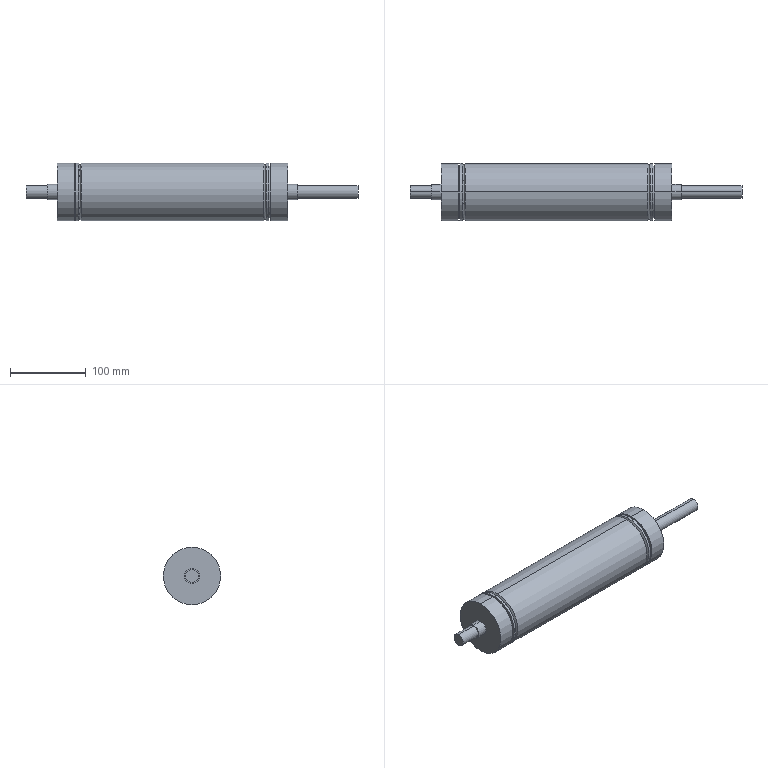Component | SolidWorks | DriveRoller-1 | 5 solids | 54 faces | box 439 x 76 x 76 mm | volume 564265 mm3 | cylinder 28 | plane 18 | cone 8 | commonest cylinder face diameters 76 x10 68 x6 70 x4 17 x4 20 x4
build123d program:
from build123d import *
from OCP.BRepFilletAPI import BRepFilletAPI_MakeChamfer

# Parameters (mm, degrees)
SKETCH1_W      = 245
SKETCH1_H      = 4
CHAMFER1_SIZE  = 3
CHAMFER1_SIZE2 = 1.732
CHAMFER2_SIZE  = 3
CHAMFER2_SIZE2 = 1.732
CHAMFER3_SIZE  = 3
CHAMFER3_SIZE2 = 1.732


with BuildPart() as part:
    # Sketch1 → Revolve1 (revolve)
    with BuildSketch(Plane.XY, mode=Mode.PRIVATE) as revolve1_sk:
        with Locations((152.5, 36)):
            Rectangle(SKETCH1_W, SKETCH1_H)
    revolve(revolve1_sk.sketch.rotate(Axis((-307.002, 0, 0), (1, 0, 0)), 90), axis=Axis((-307.002, 0, 0), (1, 0, 0)))

    # Chamfer1: one chamfer whose edges measure the first distance from different faces: ONE call of the kernel's chamfer builder (chamfer() names one face for all edges)
    chamfer1_edges_1 = [part.edges().sort_by_distance(p)[0] for p in [
        (30, 0, -38),
    ]]
    chamfer1_side_1 = [part.faces().sort_by_distance(p)[0] for p in [
        (30, 0, -36.925),
    ]]
    chamfer1_edges_2 = [part.edges().sort_by_distance(p)[0] for p in [
        (275, 0, -38),
    ]]
    chamfer1_side_2 = [part.faces().sort_by_distance(p)[0] for p in [
        (275, 0, -35.075),
    ]]
    chamfer1 = BRepFilletAPI_MakeChamfer(part.part.solid().wrapped)
    for e in chamfer1_edges_1:
        chamfer1.Add(CHAMFER1_SIZE, CHAMFER1_SIZE2, e.wrapped, chamfer1_side_1[0].wrapped)  # the first distance lies on this face
    for e in chamfer1_edges_2:
        chamfer1.Add(CHAMFER1_SIZE, CHAMFER1_SIZE2, e.wrapped, chamfer1_side_2[0].wrapped)  # the first distance lies on this face
    add(Compound.cast(chamfer1.Shape()), mode=Mode.REPLACE)


with BuildPart() as body_2:
    # Sketch2 → Revolve2 (revolve)
    with BuildSketch(Plane.XY, mode=Mode.PRIVATE) as revolve2_sk:
        Polygon((36, 0), (0, 0), (0, 38), (22.5, 38), (22.5, 35), (25, 35), (25, 38), (30, 38), (30, 34), (36, 34), align=None)
        Polygon((269, 0), (305, 0), (305, 38), (282.5, 38), (282.5, 35), (280, 35), (280, 38), (275, 38), (275, 34), (269, 34), align=None)
    revolve(revolve2_sk.sketch.rotate(Axis((-1000, 0, 0), (1, 0, 0)), 90), axis=Axis((-1000, 0, 0), (1, 0, 0)))

    # Chamfer2
    chamfer2_edges = [body_2.edges().sort_by_distance(p)[0] for p in [
        (30, 0, -38),
    ]]
    chamfer2_side = [body_2.faces().sort_by_distance(p)[0] for p in [
        (30, 0, -36.925),
    ]]
    chamfer(chamfer2_edges, length=CHAMFER2_SIZE, length2=CHAMFER2_SIZE2, reference=chamfer2_side[0])

    # Chamfer3
    chamfer3_edges = [body_2.edges().sort_by_distance(p)[0] for p in [
        (275, 0, -38),
    ]]
    chamfer3_side = [body_2.faces().sort_by_distance(p)[0] for p in [
        (275, 0, -36.925),
    ]]
    chamfer(chamfer3_edges, length=CHAMFER3_SIZE, length2=CHAMFER3_SIZE2, reference=chamfer3_side[0])


with BuildPart() as body_3:
    # Sketch3 → Revolve3 (revolve)
    with BuildSketch(Plane.XY, mode=Mode.PRIVATE) as revolve3_sk:
        Polygon((0, 10), (-13, 10), (-13, 8.5), (-41, 8.5), (-41, 0), (0, 0), align=None)
        Polygon((305, 10), (318, 10), (318, 8.5), (398, 8.5), (398, 0), (305, 0), align=None)
    revolve(revolve3_sk.sketch.rotate(Axis((-41, 0, 0), (1, 0, 0)), 90), axis=Axis((-41, 0, 0), (1, 0, 0)))


solid = Compound([part.part, body_2.part, body_3.part])

# Placed as in the assembly
solid = solid.moved(Location((5782.506, 2733.679, 47.375), (0, 0, 0)))